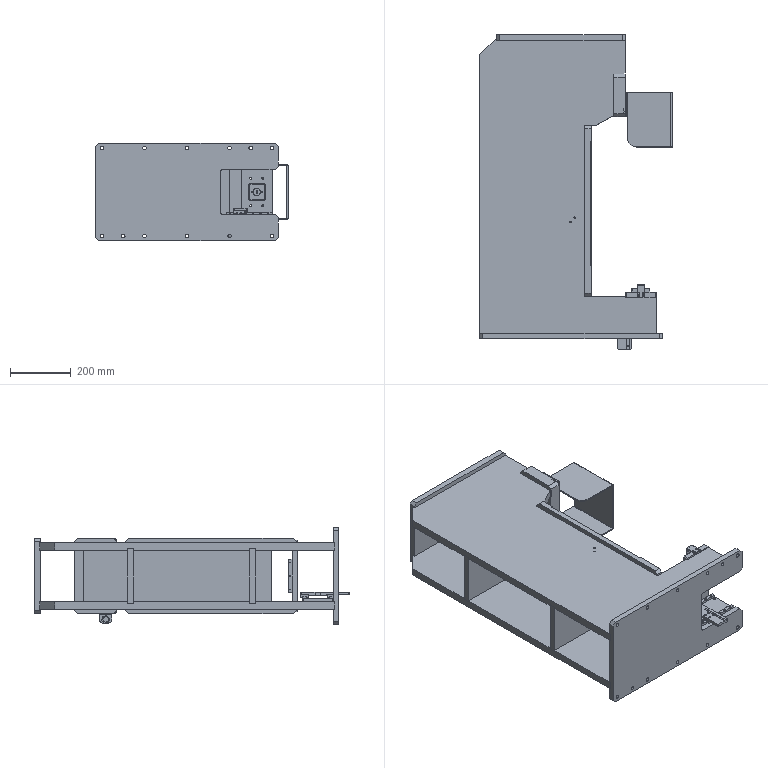Assembly | SolidWorks | mm | 22 component files | 22 solids | 1055 faces | box 633 x 1034.5 x 320 mm | volume 32101359 mm3 | cylinder 443 | plane 424 | cone 124 | spline 60 | torus 4 | commonest cylinder face diameters 6 x56 2.5 x52 3.4 x40 6.8 x32 4.2 x32 5 x22 4.5 x22 12.5 x20
Bill of materials:
000-08 | 1 | Transparent Acrylic | Thin-wall bent channel with a hat-shaped profile: a flat web, two parallel legs, and a narrower tab bent outward at the end of each leg. Each tab has two small round holes.
000-11 | 1 | 6061 | Thick L-shaped bracket. A rectangular top flange has two small through-holes near its ends. The perpendicular leg has one large central round hole and rounded lower corners.
100-01 | 1 | 45 | Flat rectangular plate with chamfered corners. A rectangular notch is open at one short end, leaving two prongs. Rows of small holes run along both long edges.
100-02 | 1 | 45 | Thin flat plate with an irregular outline: a long body with a large rectangular cutout on one side, a stepped and angled notch profile, and one chamfered corner. Two tiny holes are visible near the middle.
100-03 | 1 | 45 | Thin flat plate with the same irregular outline as unnamed part 1: a rectangular side cutout, stepped and angled notches, and one chamfered corner. It also has two lines across the top face and a few more small holes, including four near the foot end.
100-04 | 1 | 45 | Rectangular plate with chamfered corners. A shallow rebate (step) runs along each long edge on one face, ending short of the plate ends.
100-05 | 1 | 45 | Thick rectangular block with chamfered corners on its main face. Eight small holes form a symmetric pattern on the face, with stepped rebates along one side and a small rectangular notch near one end.
100-06 | 1 | 45 | Long flat plate. One end has an open U-shaped notch forming two prongs with chamfered tips; the other end has a narrower rectangular tongue. Two rows of small holes run along the length, with a thin line beside one row.
100-07 | 2 | 45 | Plain rectangular block or plate with no visible holes, chamfers, or other features.
200-02 | 1 | 6061 | Thick rectangular plate with many holes: larger holes grouped near the short ends, small holes near the corners, and a row of small shaded holes along each long edge.
200-03 | 1 | 45 | Elongated rectangular bar plate with small corner chamfers. It has several groups of round holes and an open-ended slot cut in from one long edge, plus a thin line along part of its length.
300-01 | 2 | SUS304 | L-shaped bent bracket of constant thickness with a rounded bend. One leg has two parallel elongated slots; the other leg has two round holes. Both legs have chamfered free corners.
300-02 | 1 | Cr12MoV | Rectangular plate with chamfered corners. A raised rectangular pad on one face covers the middle region. It has a large central round through hole with one small hole on each side, and three holes in a row at each end of the plate.
300-03 | 1 | Cr12MoV | Round flange disc with a smaller cylindrical boss on one side, centered on the same axis. The flange has two holes on opposite sides of the boss, and there is an elongated (obround) slot at the center of the boss.
300-05 | 1 | 45 | Long rectangular plate with chamfered corners. It has a central through cutout shaped like a square with rounded corners, four small holes around the cutout, and two pairs of larger holes at each end (eight in total). The ends are stepped thinner than the middle, and two small holes are visible in one long edge face.
M18GRYPQ | 1 | 45 | Shaft-like part that turns around a single axis, with a hexagonal collar partway along its length. On one side of the hex is a longer cylinder. On the other side is a shorter cylinder that steps down to a smaller-diameter end section.
TM12NN | 2 | 45 | Rectangular block with a rectangular channel cut across the full width of its underside, giving a bridge- or inverted-U-shaped end profile. Four round holes in a rectangular pattern enter the top face.
TM12NN-150 | 2 | 45 | Long, thin rectangular bar with six evenly spaced round holes in a single row along its length.
Mates:
1. coincident | 100-01-1 plane at (0, 0, 0) dir (0, 0, -1) | assembly plane at (0, 0, 0) dir (0, 0, 1)
2. coincident | 100-01-1 face at (0, 14, 0) dir (0, 1, 0) | 100-02-1 face at (-300, 14, 110) dir (0, -1, 0)
3. coincident | 100-01-1 face at (-300, 18, -160) dir (-1, 0, 0) | 100-02-1 face at (-300, 14, 110) dir (-1, 0, 0)
4. coincident | 100-01-1 face at (0, 14, 0) dir (0, 1, 0) | 100-03-1 face at (-300, 14, -85) dir (0, -1, 0)
5. coincident | 100-01-1 face at (-300, 18, -160) dir (-1, 0, 0) | 100-03-1 face at (-300, 14, -85) dir (-1, 0, 0)
6. distance | 100-02-1 face at (-300, 14, 110) dir (0, 0, 1) | 100-01-1 face at (300, 18, 160) dir (0, 0, 1)
7. coincident | 100-03-1 face at (-250, 984, -85) dir (0, 1, 0) | 100-04-1 face at (-33.5, 984, 0) dir (0, -1, 0)
8. width | 100-04-1 face at (-246, 1000, 125) dir (0, 0, 1) | 100-04-1 face at (-246, 1000, -125) dir (0, 0, -1) | 100-02-1 face at (-300, 14, 110) dir (0, 0, 1) | 100-03-1 face at (-300, 14, -110) dir (0, 0, -1)
9. coincident | 100-03-1 face at (179, 984, -85) dir (1, 0, 0) | 100-04-1 face at (179, 1000, 125) dir (1, 0, 0)
10. coincident | 100-02-1 face at (179, 871, 110) dir (0, -1, 0) | 100-05-1 face at (179, 871, -125) dir (0, 1, 0)
11. width | 100-05-1 face at (179, 871, -125) dir (0, 0, -1) | 100-05-1 face at (179, 871, 125) dir (0, 0, 1) | 100-02-1 face at (-300, 14, 110) dir (0, 0, 1) | 100-03-1 face at (-300, 14, -110) dir (0, 0, -1)
12. width | 100-06-1 face at (66, 140, 125) dir (0, 0, 1) | 100-06-1 face at (66, 140, -125) dir (0, 0, -1) | 100-03-1 face at (-300, 14, -110) dir (0, 0, -1) | 100-02-1 face at (-300, 14, 110) dir (0, 0, 1)
13. coincident | 100-02-1 face at (50, 701, 110) dir (0, -1, 0) | 100-06-1 face at (46, 701, 125) dir (0, 1, 0)
14. coincident | 100-03-1 face at (-300, 14, -85) dir (-1, 0, 0) | 100-07-1 face at (-300, 294, 89) dir (-1, 0, 0)
15. coincident | 100-02-1 face at (-300, 14, 110) dir (-1, 0, 0) | 100-07-2 face at (-300, 694, 89) dir (-1, 0, 0)
16. coincident | 100-03-1 face at (145, 871, -85) dir (1, 0, 0) | 100-05-1 face at (145, 801, 0) dir (-1, 0, 0)
17. coincident | 100-03-1 face at (50, 140, -85) dir (1, 0, 0) | 100-06-1 face at (50, 490, 0) dir (-1, 0, 0)
18. width | 100-07-2 face at (-127, 694, 0) dir (0, 1, 0) | 100-07-2 face at (-127, 674, 0) dir (0, -1, 0) | 100-03-1 face at (-300, 694, -89) dir (0, -1, 0) | 100-03-1 face at (-300, 674, -89) dir (0, 1, 0)
19. coincident | 100-03-1 face at (-300, 414, -89) dir (0, 0, 1) | 100-07-2 face at (-300, 694, -89) dir (0, 0, -1)
20. coincident | 100-03-1 face at (-300, 274, -89) dir (0, 1, 0) | 100-07-1 face at (-127, 274, 0) dir (0, -1, 0)
21. coincident | 100-03-1 face at (-300, 14, -89) dir (0, 0, 1) | 100-07-1 face at (-300, 294, -89) dir (0, 0, -1)
22. concentric | 100-05-1 face at (179, 799, -110) dir (1, 0, 0) r 3.4 | 000-08-1 face at (179, 799, -110) dir (1, 0, 0) r 4.25
23. concentric | 100-05-1 face at (179, 771, -110) dir (1, 0, 0) r 3.4 | 000-08-1 face at (179, 771, -110) dir (1, 0, 0) r 4.25
24. coincident | 100-05-1 face at (179, 801, 0) dir (1, 0, 0) | 000-08-1 face at (179, 811, -92.5) dir (-1, 0, 0)
25. coincident | 100-01-1 face at (0, 18, 0) dir (0, 1, 0) | 200-02-1 face at (100, 18, -75) dir (0, -1, 0)
26. coincident | 100-03-1 face at (-300, 14, -85) dir (0, 0, 1) | 200-02-1 face at (190, 68, -85) dir (0, 0, -1)
27. coincident | 100-03-1 face at (280, 14, -85) dir (1, 0, 0) | 200-02-1 face at (280, 18, -75) dir (1, 0, 0)
28. coincident | 200-02-1 face at (190, 68, -75) dir (0, 0, 1) | TM12NNA-1-150-NA-Z0-1/TM12NN-150-1 face at (280, 18, -75) dir (0, 0, -1)
29. concentric | 200-02-1 face at (267.5, 24, -75) dir (0, 0, 1) r 1.25 | TM12NNA-1-150-NA-Z0-1/TM12NN-150-1 face at (267.5, 24, -67.5) dir (0, 0, 1) r 1.7
30. concentric | 200-02-1 face at (167.5, 24, -75) dir (0, 0, 1) r 1.25 | TM12NNA-1-150-NA-Z0-1/TM12NN-150-1 face at (167.5, 24, -67.5) dir (0, 0, 1) r 1.7
31. coincident | 200-02-1 face at (190, 68, -75) dir (0, 0, 1) | TM12NNA-1-150-NA-Z0-2/TM12NN-150-1 face at (280, 106, -75) dir (0, 0, -1)
32. concentric | 200-02-1 face at (267.5, 112, -75) dir (0, 0, 1) r 1.25 | TM12NNA-1-150-NA-Z0-2/TM12NN-150-1 face at (267.5, 112, -67.5) dir (0, 0, 1) r 1.7
33. concentric | 200-02-1 face at (192.5, 112, -75) dir (0, 0, 1) r 1.25 | TM12NNA-1-150-NA-Z0-2/TM12NN-150-1 face at (192.5, 112, -67.5) dir (0, 0, 1) r 1.7
34. coincident | TM12NNA-1-150-NA-Z0-1/TM12NN-1 face at (188.8, 37.5, -72) dir (1, 0, 0) | TM12NNA-1-150-NA-Z0-2/TM12NN-1 face at (188.8, 125.5, -72) dir (1, 0, 0)
35. coincident | TM12NNA-1-150-NA-Z0-2/TM12NN-1 face at (171.3, 112, -62) dir (0, 0, 1) | 200-03-1 face at (176.3, 45.5, -62) dir (0, 0, -1)
36. concentric | TM12NNA-1-150-NA-Z0-2/TM12NN-1 face at (178.8, 122, -62) dir (0, 0, 1) r 1.25 | 200-03-1 face at (178.8, 122, -53) dir (0, 0, 1) r 1.7
37. coincident | 100-03-1 face at (280, 140, -85) dir (0, 1, 0) | 300-05-1 face at (230, 140, 0) dir (0, -1, 0)
38. concentric | 100-03-1 face at (252.5, 140, -97.5) dir (0, 1, 0) r 3.4 | 300-05-1 face at (252.5, 153, -97.5) dir (0, 1, 0) r 4.5
39. concentric | 100-03-1 face at (207.5, 140, -97.5) dir (0, 1, 0) r 3.4 | 300-05-1 face at (207.5, 153, -97.5) dir (0, 1, 0) r 4.5
40. coincident | 300-02-1 face at (230, 153, 0) dir (0, -1, 0) | 300-05-1 face at (230, 153, 0) dir (0, 1, 0)
41. concentric | 300-02-1 face at (250, 165, -45) dir (0, 1, 0) r 4.5 | 300-05-1 face at (250, 153, -45) dir (0, 1, 0) r 3.4
42. concentric | 300-02-1 face at (210, 165, -45) dir (0, 1, 0) r 4.5 | 300-05-1 face at (210, 153, -45) dir (0, 1, 0) r 3.4
43. coincident | 300-05-1 face at (180, 135, 115) dir (0, 0, 1) | 300-01-1 face at (242.5, 175, 115) dir (0, 0, -1)
44. coincident | 300-05-1 face at (230, 135, 0) dir (0, -1, 0) | 300-01-1 face at (242.5, 135, 115) dir (0, -1, 0)
45. coincident | 300-05-1 face at (180, 135, -115) dir (0, 0, -1) | 300-01-2 face at (217.5, 175, -115) dir (0, 0, 1)
46. width | 300-01-2 face at (224.75, 140, -118) dir (-1, 0, 0) | 300-01-2 face at (220.25, 140, -118) dir (1, 0, 0) | 300-05-1 face at (222.5, 145, -115) dir (0, 0, -1) r 1.65
47. width | 300-01-2 face at (235.25, 140, -118) dir (1, 0, 0) | 300-01-2 face at (239.75, 140, -118) dir (-1, 0, 0) | 300-05-1 face at (237.5, 145, -115) dir (0, 0, -1) r 1.65
48. coincident | 300-05-1 face at (230, 135, 0) dir (0, -1, 0) | 300-01-2 face at (217.5, 135, -115) dir (0, -1, 0)
49. coincident | 300-01-2 face at (242.5, 175, -115) dir (1, 0, 0) | 300-01-1 face at (242.5, 175, 115) dir (1, 0, 0)
50. coincident | 100-05-1 face at (179, 871, -125) dir (0, 0, -1) | 000-11-1 face at (179, 787, -125) dir (0, 0, 1)
51. concentric | 100-05-1 face at (169, 783, -125) dir (0, 0, -1) r 1.25 | 000-11-1 face at (169, 783, -128) dir (0, 0, -1) r 2.25
52. concentric | 100-05-1 face at (169, 751, -125) dir (0, 0, -1) r 1.25 | 000-11-1 face at (169, 751, -128) dir (0, 0, -1) r 2.25
53. concentric | 000-11-1 face at (164, 767, -143) dir (1, 0, 0) r 9.5 | M18GRYPQ-1 face at (137, 767, -143) dir (1, 0, 0) r 9
54. coincident | 000-11-1 face at (176, 747, -155) dir (-1, 0, 0) | M18GRYPQ-1 face at (176, 767, -143) dir (1, 0, 0)
55. concentric | 300-02-1 face at (230, 148, 0) dir (0, 1, 0) r 12.5 | 300-03-1 face at (230, 148, 0) dir (0, 1, 0) r 12.5
56. coincident | 300-02-1 face at (230, 156, 0) dir (0, 1, 0) | 300-03-1 face at (230, 156, 0) dir (0, -1, 0)
57. coincident | TM12NN-150-1 face at (89.369, 88.252, 154.936) dir (0, 1, 0) | TM12NN-1 face at (101.369, 88.252, 28.736) dir (0, -1, 0)
58. width | TM12NN-1 face at (81.869, 83.752, 28.736) dir (-1, 0, 0) | TM12NN-1 face at (108.869, 83.752, 28.736) dir (1, 0, 0) | TM12NN-150-1 face at (101.369, 80.752, 154.936) dir (1, 0, 0) | TM12NN-150-1 face at (89.369, 80.752, 154.936) dir (-1, 0, 0)